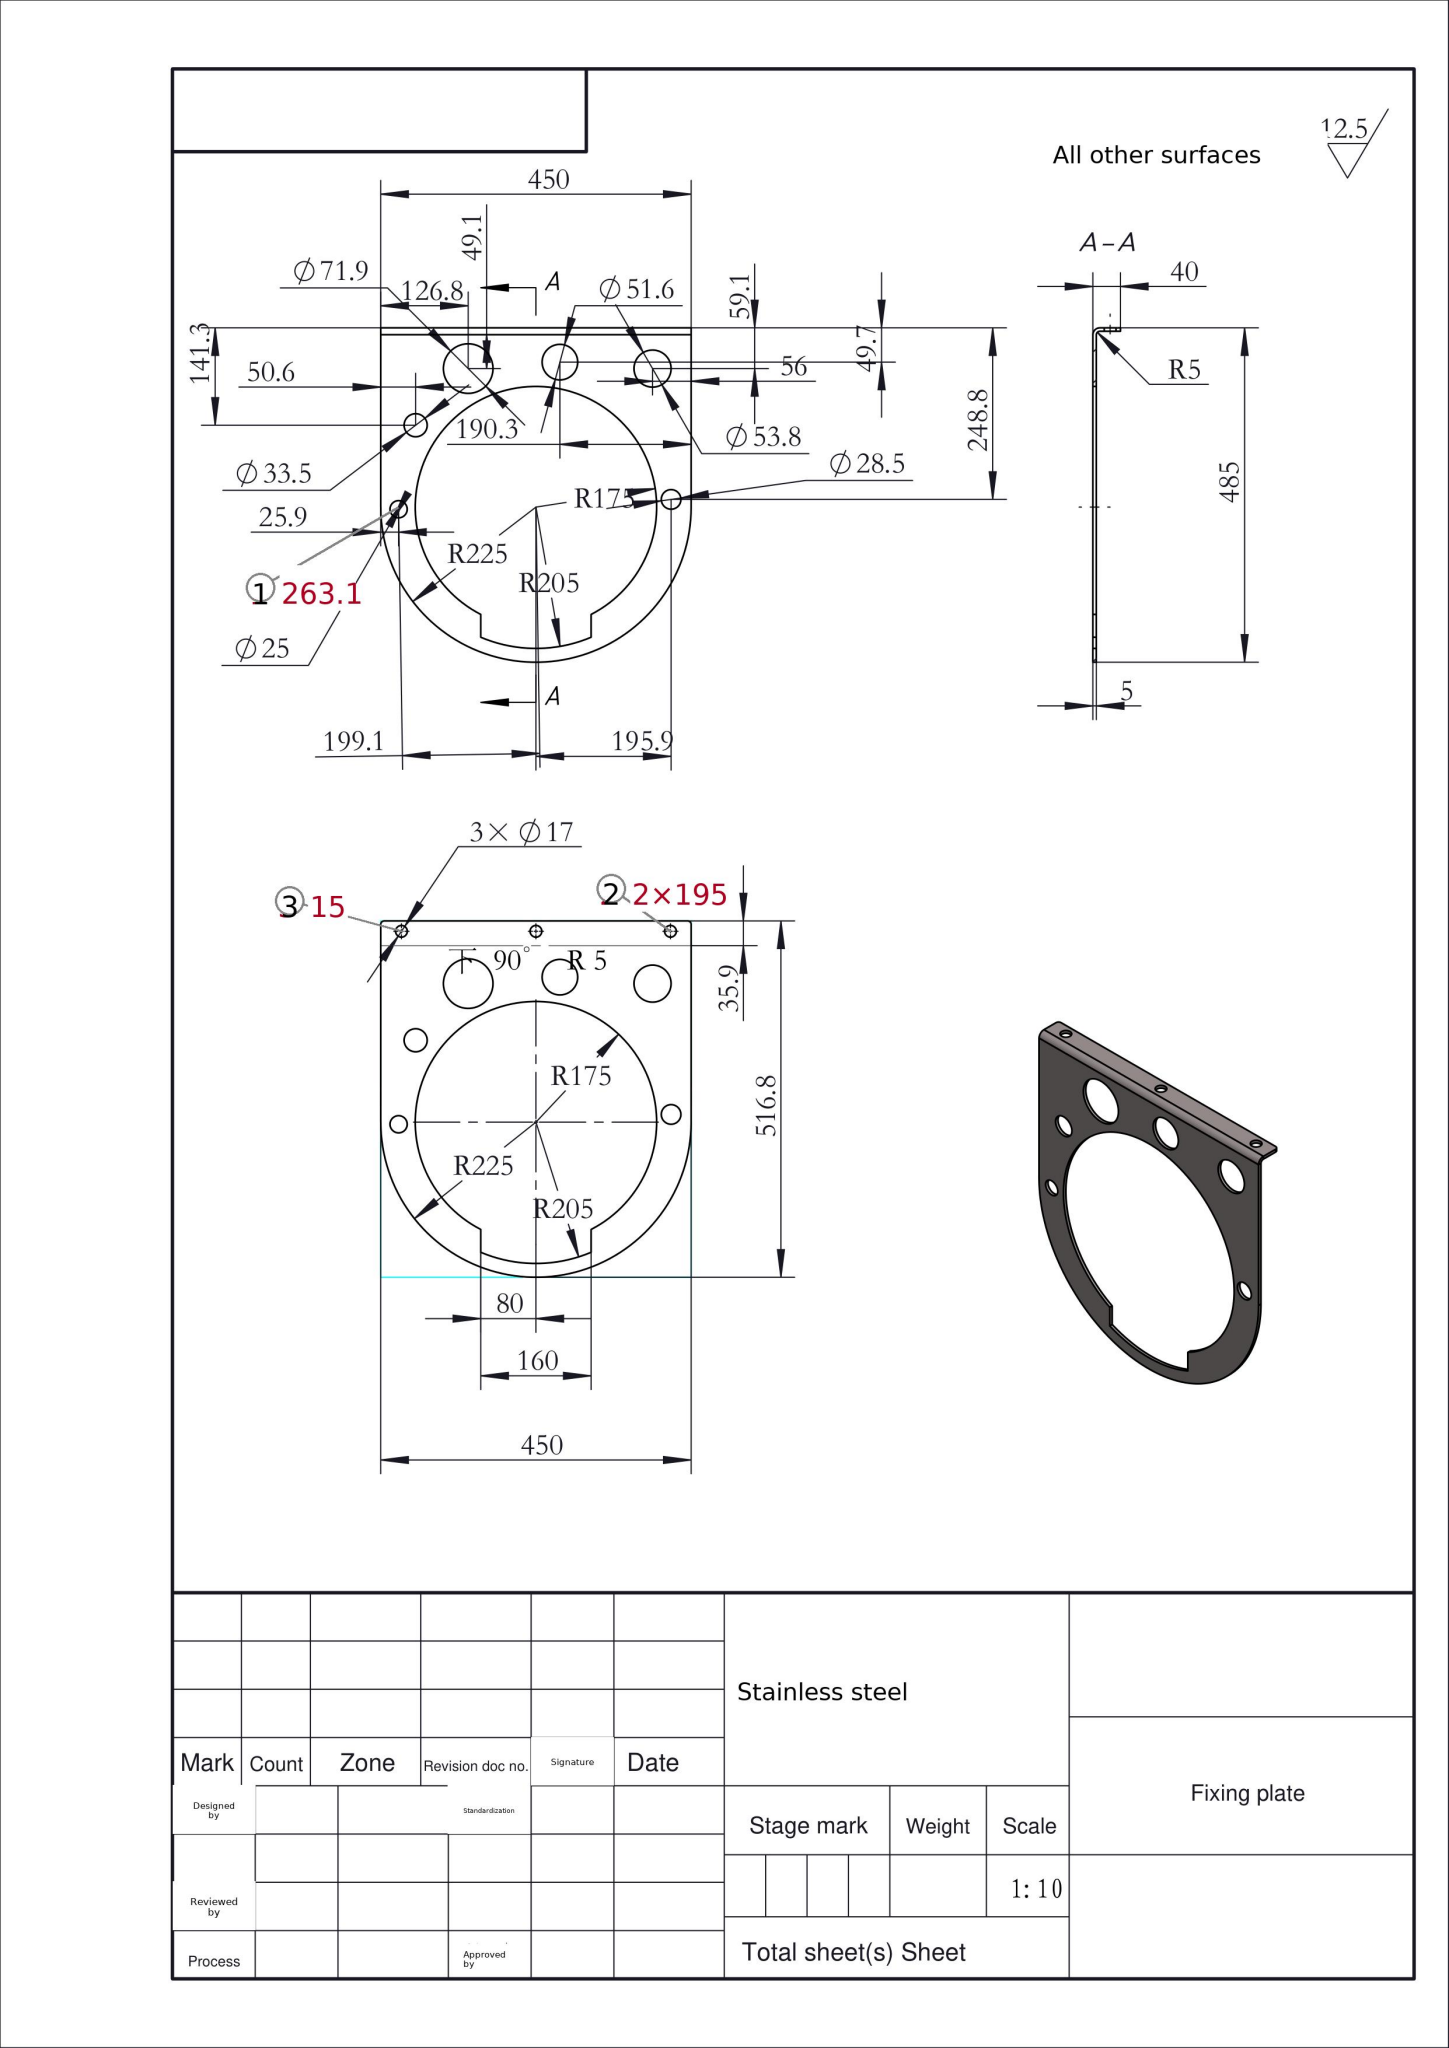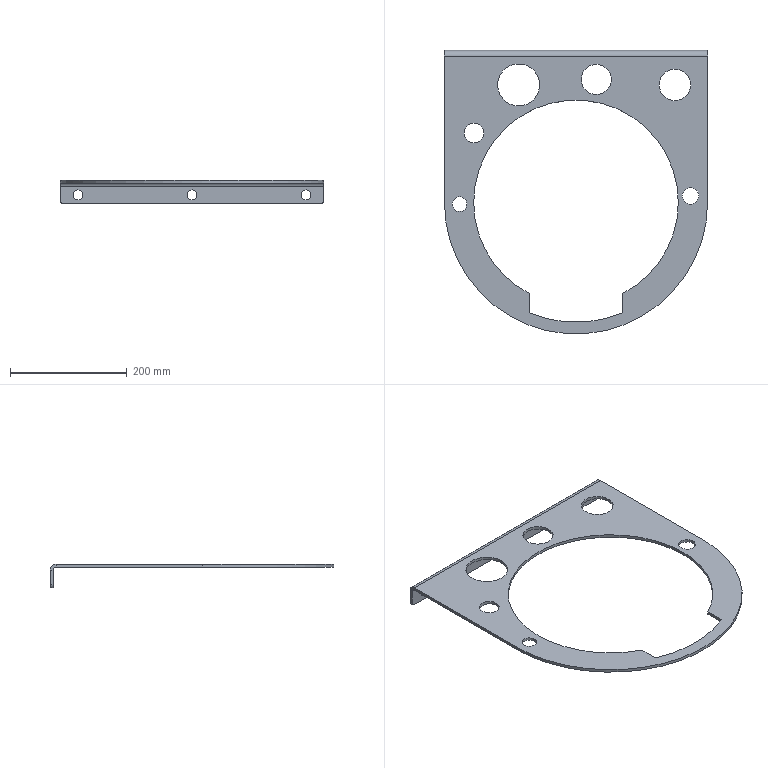Part | SolidWorks | mm | material Stainless steel | 1 solid | 40 faces | box 450 x 485 x 40 mm | volume 492630 mm3 | cylinder 27 | plane 13 | commonest cylinder face diameters 17 x6 350 x3 10 x3 51.615 x2 71.923 x2 33.513 x2 28.488 x2 24.989 x2